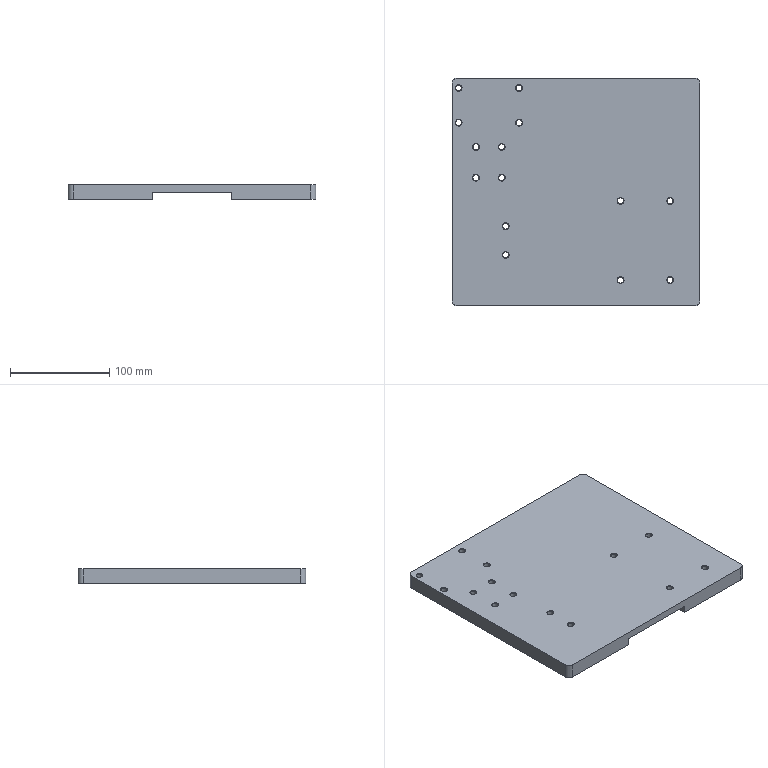Component | NX | BASE | 1 solid | 56 faces | volume 718171 mm3 | cone 28 | cylinder 18 | plane 10 | commonest cylinder face diameters 6 x14 10 x4